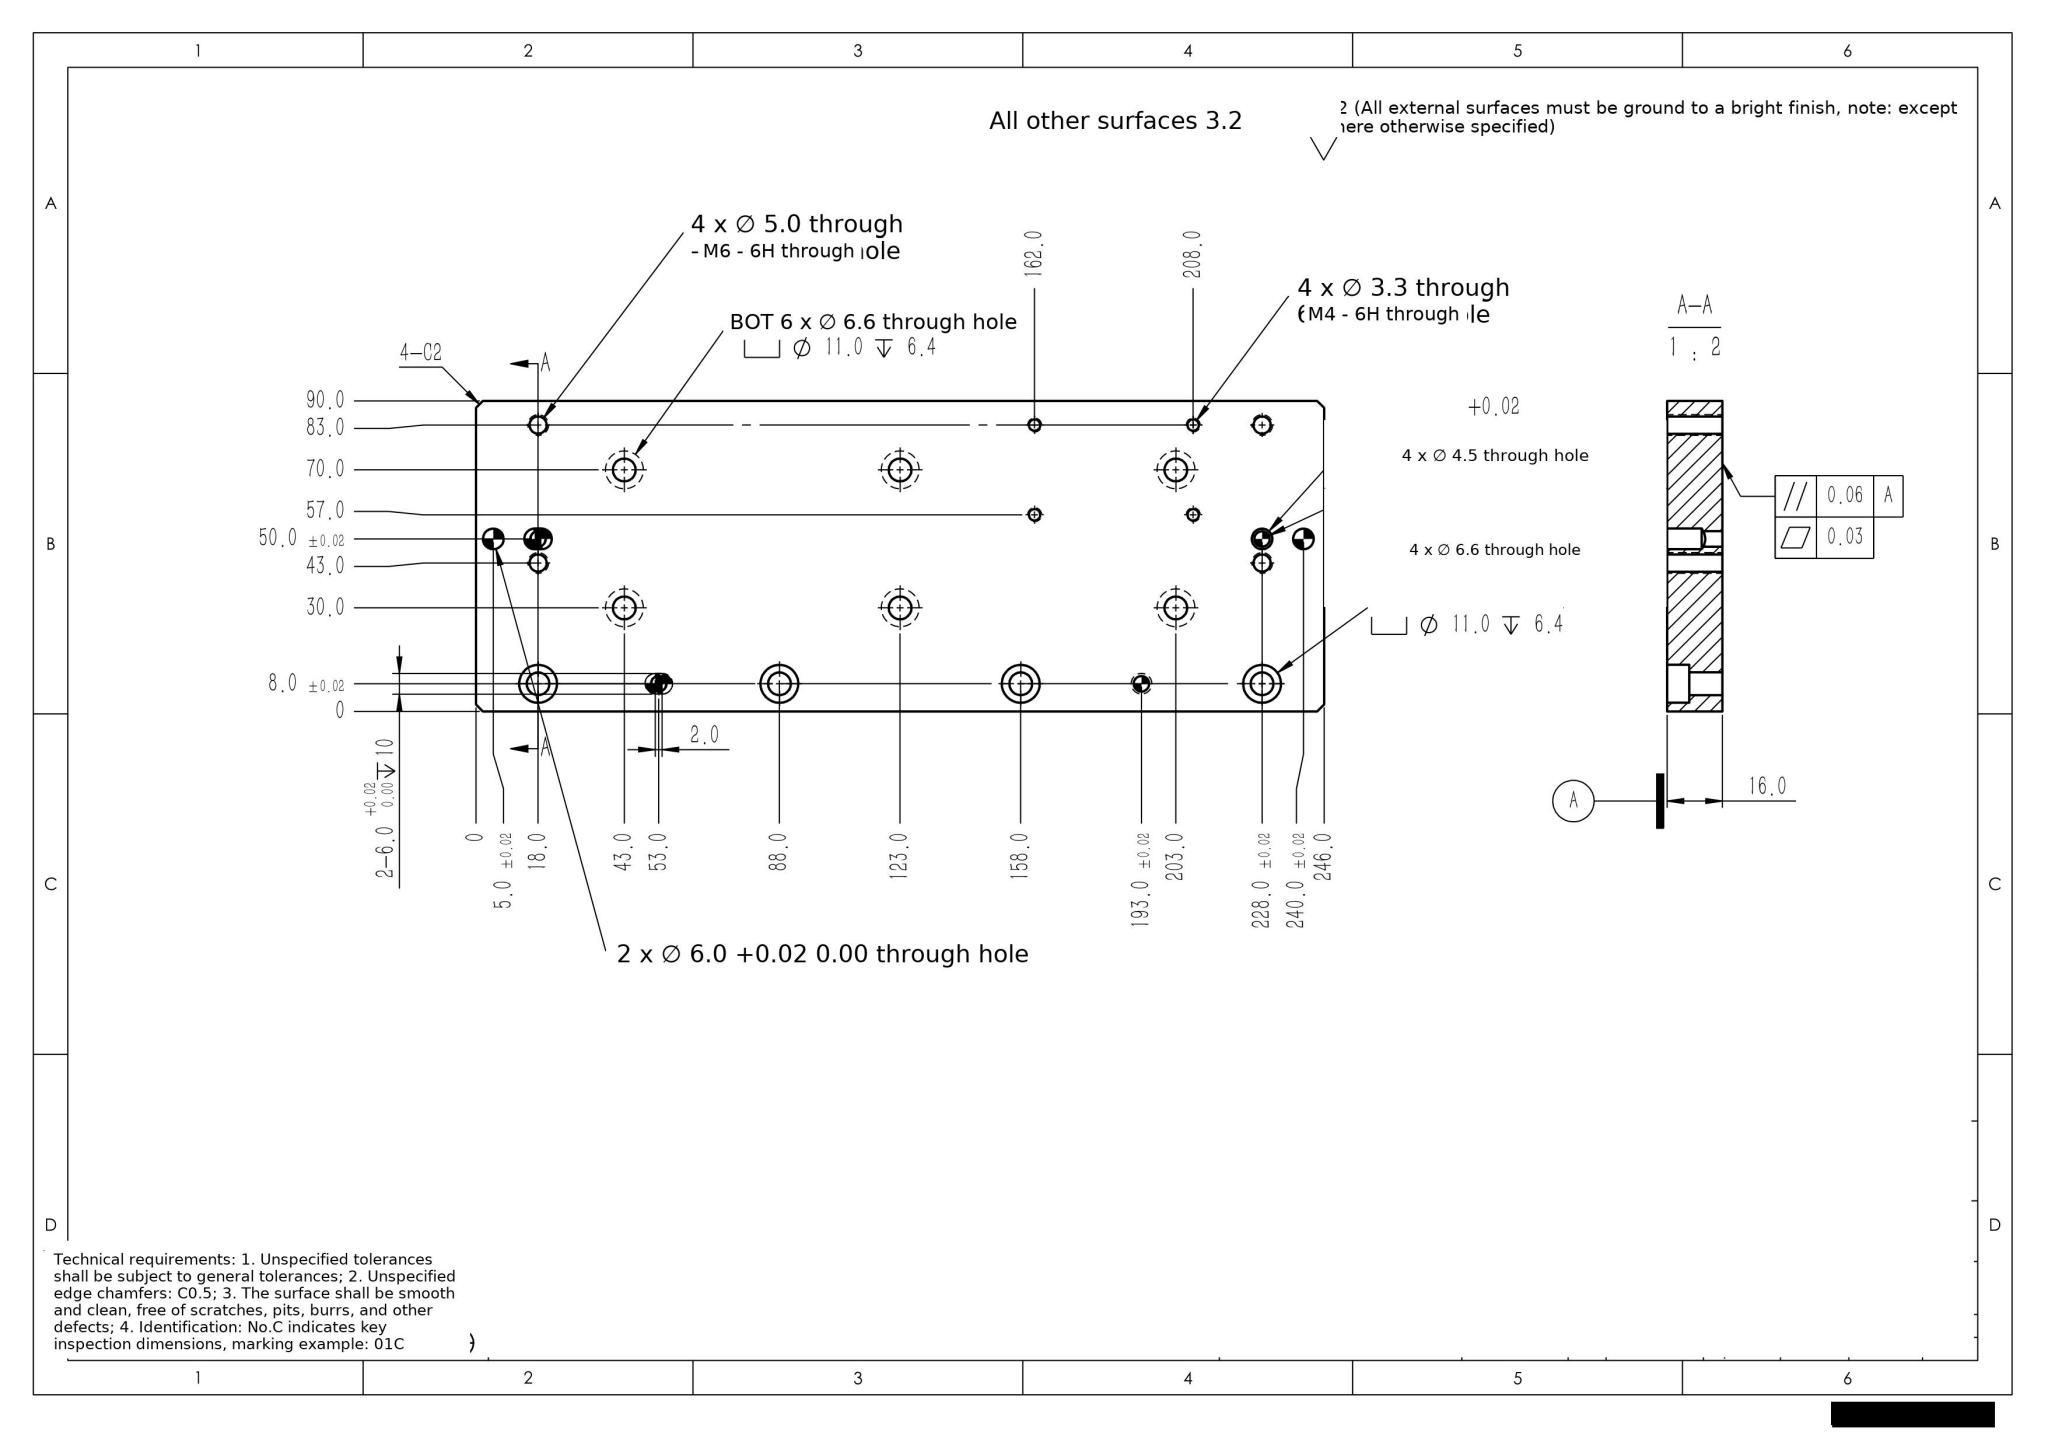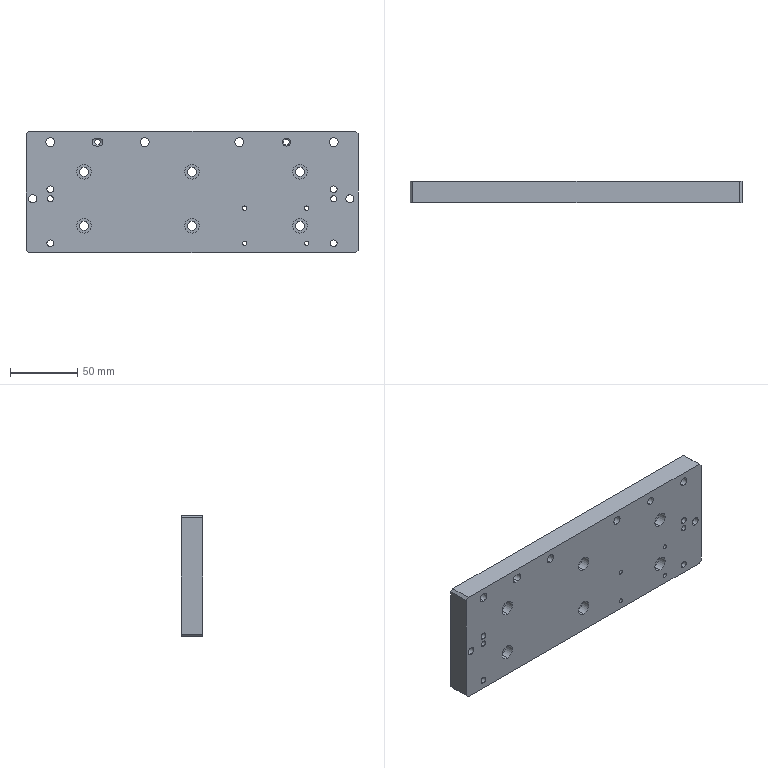Part | SolidWorks | mm | 1 solid | 112 faces | box 246 x 16 x 90 mm | volume 340352 mm3 | cylinder 76 | plane 28 | cone 8 | commonest cylinder face diameters 11 x20 6.6 x20 6 x12 3.3 x8 5 x8 4.5 x8